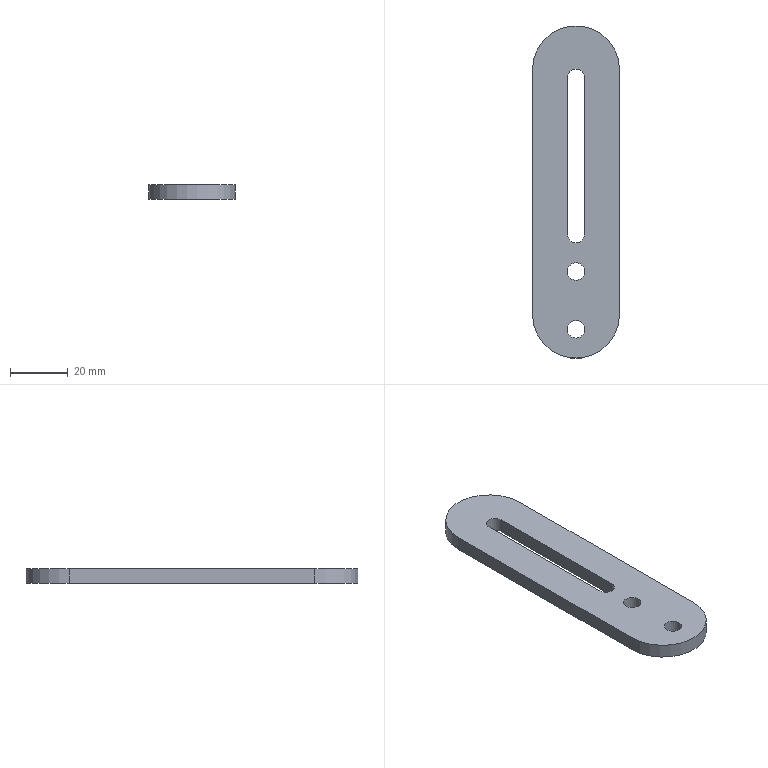Component | NX | BALL_HEAD_WAIST_PLATE | 1 solid | 12 faces | box 30 x 115 x 5 mm | volume 14240 mm3 | plane 6 | cylinder 6 | commonest cylinder face diameters 6 x4 30 x2
STEP:
#1=CARTESIAN_POINT('',(0.,0.,0.));
#2=DIRECTION('',(0.,0.,1.));
#3=DIRECTION('',(1.,0.,0.));
#4=AXIS2_PLACEMENT_3D('',#1,#2,#3);
#5=CARTESIAN_POINT('',(-63.,-45.593,2.5));
#6=VERTEX_POINT('',#5);
#7=CARTESIAN_POINT('',(-63.,8.407,2.5));
#8=VERTEX_POINT('',#7);
#9=CARTESIAN_POINT('',(-63.,-48.593,2.5));
#10=DIRECTION('',(0.,1.,0.));
#11=VECTOR('',#10,1.);
#12=LINE('',#9,#11);
#13=CARTESIAN_POINT('',(-63.,-48.593,7.5));
#14=DIRECTION('',(-1.,0.,0.));
#15=DIRECTION('',(0.,0.,-1.));
#16=AXIS2_PLACEMENT_3D('',#13,#14,#15);
#17=PLANE('',#16);
#18=CARTESIAN_POINT('',(5.,0.));
#19=DIRECTION('',(0.,-1.));
#20=VECTOR('',#19,1.);
#21=LINE('',#18,#20);
#22=(GEOMETRIC_REPRESENTATION_CONTEXT(2)PARAMETRIC_REPRESENTATION_CONTEXT()REPRESENTATION_CONTEXT('',''));
#23=DEFINITIONAL_REPRESENTATION('',(#21),#22);
#24=PCURVE('',#17,#23);
#25=CARTESIAN_POINT('',(-60.,-78.593,2.5));
#26=DIRECTION('',(0.,0.,1.));
#27=DIRECTION('',(0.,-1.,0.));
#28=AXIS2_PLACEMENT_3D('',#25,#26,#27);
#29=PLANE('',#28);
#30=CARTESIAN_POINT('',(-30.,-3.));
#31=DIRECTION('',(-1.,0.));
#32=VECTOR('',#31,1.);
#33=LINE('',#30,#32);
#34=(GEOMETRIC_REPRESENTATION_CONTEXT(2)PARAMETRIC_REPRESENTATION_CONTEXT()REPRESENTATION_CONTEXT('',''));
#35=DEFINITIONAL_REPRESENTATION('',(#33),#34);
#36=PCURVE('',#29,#35);
#37=SURFACE_CURVE('',#12,(#24,#36),.PCURVE_S1.);
#38=EDGE_CURVE('',#6,#8,#37,.T.);
#39=ORIENTED_EDGE('',*,*,#38,.T.);
#40=CARTESIAN_POINT('',(-63.,8.407,7.5));
#41=VERTEX_POINT('',#40);
#42=CARTESIAN_POINT('',(-63.,8.407,7.5));
#43=DIRECTION('',(0.,0.,1.));
#44=VECTOR('',#43,1.);
#45=LINE('',#42,#44);
#46=CARTESIAN_POINT('',(0.,-57.));
#47=DIRECTION('',(-1.,0.));
#48=VECTOR('',#47,1.);
#49=LINE('',#46,#48);
#50=(GEOMETRIC_REPRESENTATION_CONTEXT(2)PARAMETRIC_REPRESENTATION_CONTEXT()REPRESENTATION_CONTEXT('',''));
#51=DEFINITIONAL_REPRESENTATION('',(#49),#50);
#52=PCURVE('',#17,#51);
#53=CARTESIAN_POINT('',(-60.,8.407,7.5));
#54=DIRECTION('',(0.,0.,1.));
#55=DIRECTION('',(0.,-1.,0.));
#56=AXIS2_PLACEMENT_3D('',#53,#54,#55);
#57=CYLINDRICAL_SURFACE('',#56,3.);
#58=CARTESIAN_POINT('',(4.712,0.));
#59=DIRECTION('',(0.,1.));
#60=VECTOR('',#59,1.);
#61=LINE('',#58,#60);
#62=(GEOMETRIC_REPRESENTATION_CONTEXT(2)PARAMETRIC_REPRESENTATION_CONTEXT()REPRESENTATION_CONTEXT('',''));
#63=DEFINITIONAL_REPRESENTATION('',(#61),#62);
#64=PCURVE('',#57,#63);
#65=SURFACE_CURVE('',#45,(#52,#64),.PCURVE_S1.);
#66=EDGE_CURVE('',#8,#41,#65,.T.);
#67=ORIENTED_EDGE('',*,*,#66,.T.);
#68=CARTESIAN_POINT('',(-63.,-45.593,7.5));
#69=VERTEX_POINT('',#68);
#70=CARTESIAN_POINT('',(-63.,-48.593,7.5));
#71=DIRECTION('',(0.,1.,0.));
#72=VECTOR('',#71,1.);
#73=LINE('',#70,#72);
#74=CARTESIAN_POINT('',(0.,0.));
#75=DIRECTION('',(0.,-1.));
#76=VECTOR('',#75,1.);
#77=LINE('',#74,#76);
#78=(GEOMETRIC_REPRESENTATION_CONTEXT(2)PARAMETRIC_REPRESENTATION_CONTEXT()REPRESENTATION_CONTEXT('',''));
#79=DEFINITIONAL_REPRESENTATION('',(#77),#78);
#80=PCURVE('',#17,#79);
#81=CARTESIAN_POINT('',(-60.,-78.593,7.5));
#82=DIRECTION('',(0.,0.,1.));
#83=DIRECTION('',(0.,-1.,0.));
#84=AXIS2_PLACEMENT_3D('',#81,#82,#83);
#85=PLANE('',#84);
#86=CARTESIAN_POINT('',(-30.,-3.));
#87=DIRECTION('',(-1.,0.));
#88=VECTOR('',#87,1.);
#89=LINE('',#86,#88);
#90=(GEOMETRIC_REPRESENTATION_CONTEXT(2)PARAMETRIC_REPRESENTATION_CONTEXT()REPRESENTATION_CONTEXT('',''));
#91=DEFINITIONAL_REPRESENTATION('',(#89),#90);
#92=PCURVE('',#85,#91);
#93=SURFACE_CURVE('',#73,(#80,#92),.PCURVE_S1.);
#94=EDGE_CURVE('',#69,#41,#93,.T.);
#95=ORIENTED_EDGE('',*,*,#94,.F.);
#96=CARTESIAN_POINT('',(-63.,-45.593,2.5));
#97=DIRECTION('',(0.,0.,-1.));
#98=VECTOR('',#97,1.);
#99=LINE('',#96,#98);
#100=CARTESIAN_POINT('',(5.,-3.));
#101=DIRECTION('',(1.,0.));
#102=VECTOR('',#101,1.);
#103=LINE('',#100,#102);
#104=(GEOMETRIC_REPRESENTATION_CONTEXT(2)PARAMETRIC_REPRESENTATION_CONTEXT()REPRESENTATION_CONTEXT('',''));
#105=DEFINITIONAL_REPRESENTATION('',(#103),#104);
#106=PCURVE('',#17,#105);
#107=CARTESIAN_POINT('',(-60.,-45.593,7.5));
#108=DIRECTION('',(0.,0.,1.));
#109=DIRECTION('',(0.,-1.,0.));
#110=AXIS2_PLACEMENT_3D('',#107,#108,#109);
#111=CYLINDRICAL_SURFACE('',#110,3.);
#112=CARTESIAN_POINT('',(4.712,-5.));
#113=DIRECTION('',(0.,-1.));
#114=VECTOR('',#113,1.);
#115=LINE('',#112,#114);
#116=(GEOMETRIC_REPRESENTATION_CONTEXT(2)PARAMETRIC_REPRESENTATION_CONTEXT()REPRESENTATION_CONTEXT('',''));
#117=DEFINITIONAL_REPRESENTATION('',(#115),#116);
#118=PCURVE('',#111,#117);
#119=SURFACE_CURVE('',#99,(#106,#118),.PCURVE_S1.);
#120=EDGE_CURVE('',#69,#6,#119,.T.);
#121=ORIENTED_EDGE('',*,*,#120,.T.);
#122=EDGE_LOOP('',(#39,#67,#95,#121));
#123=FACE_BOUND('',#122,.T.);
#124=ADVANCED_FACE('',(#123),#17,.F.);
#125=CARTESIAN_POINT('',(-45.,11.407,2.5));
#126=VERTEX_POINT('',#125);
#127=CARTESIAN_POINT('',(-45.,-73.593,2.5));
#128=VERTEX_POINT('',#127);
#129=CARTESIAN_POINT('',(-45.,26.407,2.5));
#130=DIRECTION('',(0.,-1.,0.));
#131=VECTOR('',#130,1.);
#132=LINE('',#129,#131);
#133=CARTESIAN_POINT('',(-45.,26.407,7.5));
#134=DIRECTION('',(1.,0.,0.));
#135=DIRECTION('',(0.,0.,1.));
#136=AXIS2_PLACEMENT_3D('',#133,#134,#135);
#137=PLANE('',#136);
#138=CARTESIAN_POINT('',(-5.,0.));
#139=DIRECTION('',(0.,1.));
#140=VECTOR('',#139,1.);
#141=LINE('',#138,#140);
#142=(GEOMETRIC_REPRESENTATION_CONTEXT(2)PARAMETRIC_REPRESENTATION_CONTEXT()REPRESENTATION_CONTEXT('',''));
#143=DEFINITIONAL_REPRESENTATION('',(#141),#142);
#144=PCURVE('',#137,#143);
#145=CARTESIAN_POINT('',(-105.,15.));
#146=DIRECTION('',(1.,0.));
#147=VECTOR('',#146,1.);
#148=LINE('',#145,#147);
#149=(GEOMETRIC_REPRESENTATION_CONTEXT(2)PARAMETRIC_REPRESENTATION_CONTEXT()REPRESENTATION_CONTEXT('',''));
#150=DEFINITIONAL_REPRESENTATION('',(#148),#149);
#151=PCURVE('',#29,#150);
#152=SURFACE_CURVE('',#132,(#144,#151),.PCURVE_S1.);
#153=EDGE_CURVE('',#126,#128,#152,.T.);
#154=ORIENTED_EDGE('',*,*,#153,.F.);
#155=CARTESIAN_POINT('',(-45.,11.407,7.5));
#156=VERTEX_POINT('',#155);
#157=CARTESIAN_POINT('',(-45.,11.407,7.5));
#158=DIRECTION('',(0.,0.,1.));
#159=VECTOR('',#158,1.);
#160=LINE('',#157,#159);
#161=CARTESIAN_POINT('',(0.,15.));
#162=DIRECTION('',(1.,0.));
#163=VECTOR('',#162,1.);
#164=LINE('',#161,#163);
#165=(GEOMETRIC_REPRESENTATION_CONTEXT(2)PARAMETRIC_REPRESENTATION_CONTEXT()REPRESENTATION_CONTEXT('',''));
#166=DEFINITIONAL_REPRESENTATION('',(#164),#165);
#167=PCURVE('',#137,#166);
#168=CARTESIAN_POINT('',(-60.,11.407,7.5));
#169=DIRECTION('',(0.,0.,-1.));
#170=DIRECTION('',(0.,1.,0.));
#171=AXIS2_PLACEMENT_3D('',#168,#169,#170);
#172=CYLINDRICAL_SURFACE('',#171,15.);
#173=CARTESIAN_POINT('',(7.854,0.));
#174=DIRECTION('',(0.,-1.));
#175=VECTOR('',#174,1.);
#176=LINE('',#173,#175);
#177=(GEOMETRIC_REPRESENTATION_CONTEXT(2)PARAMETRIC_REPRESENTATION_CONTEXT()REPRESENTATION_CONTEXT('',''));
#178=DEFINITIONAL_REPRESENTATION('',(#176),#177);
#179=PCURVE('',#172,#178);
#180=SURFACE_CURVE('',#160,(#167,#179),.PCURVE_S1.);
#181=EDGE_CURVE('',#126,#156,#180,.T.);
#182=ORIENTED_EDGE('',*,*,#181,.T.);
#183=CARTESIAN_POINT('',(-45.,-73.593,7.5));
#184=VERTEX_POINT('',#183);
#185=CARTESIAN_POINT('',(-45.,26.407,7.5));
#186=DIRECTION('',(0.,-1.,0.));
#187=VECTOR('',#186,1.);
#188=LINE('',#185,#187);
#189=CARTESIAN_POINT('',(0.,0.));
#190=DIRECTION('',(0.,1.));
#191=VECTOR('',#190,1.);
#192=LINE('',#189,#191);
#193=(GEOMETRIC_REPRESENTATION_CONTEXT(2)PARAMETRIC_REPRESENTATION_CONTEXT()REPRESENTATION_CONTEXT('',''));
#194=DEFINITIONAL_REPRESENTATION('',(#192),#193);
#195=PCURVE('',#137,#194);
#196=CARTESIAN_POINT('',(-105.,15.));
#197=DIRECTION('',(1.,0.));
#198=VECTOR('',#197,1.);
#199=LINE('',#196,#198);
#200=(GEOMETRIC_REPRESENTATION_CONTEXT(2)PARAMETRIC_REPRESENTATION_CONTEXT()REPRESENTATION_CONTEXT('',''));
#201=DEFINITIONAL_REPRESENTATION('',(#199),#200);
#202=PCURVE('',#85,#201);
#203=SURFACE_CURVE('',#188,(#195,#202),.PCURVE_S1.);
#204=EDGE_CURVE('',#156,#184,#203,.T.);
#205=ORIENTED_EDGE('',*,*,#204,.T.);
#206=CARTESIAN_POINT('',(-45.,-73.593,7.5));
#207=DIRECTION('',(0.,0.,-1.));
#208=VECTOR('',#207,1.);
#209=LINE('',#206,#208);
#210=CARTESIAN_POINT('',(0.,100.));
#211=DIRECTION('',(-1.,0.));
#212=VECTOR('',#211,1.);
#213=LINE('',#210,#212);
#214=(GEOMETRIC_REPRESENTATION_CONTEXT(2)PARAMETRIC_REPRESENTATION_CONTEXT()REPRESENTATION_CONTEXT('',''));
#215=DEFINITIONAL_REPRESENTATION('',(#213),#214);
#216=PCURVE('',#137,#215);
#217=CARTESIAN_POINT('',(-60.,-73.593,7.5));
#218=DIRECTION('',(0.,0.,-1.));
#219=DIRECTION('',(0.,1.,0.));
#220=AXIS2_PLACEMENT_3D('',#217,#218,#219);
#221=CYLINDRICAL_SURFACE('',#220,15.);
#222=CARTESIAN_POINT('',(1.571,0.));
#223=DIRECTION('',(0.,1.));
#224=VECTOR('',#223,1.);
#225=LINE('',#222,#224);
#226=(GEOMETRIC_REPRESENTATION_CONTEXT(2)PARAMETRIC_REPRESENTATION_CONTEXT()REPRESENTATION_CONTEXT('',''));
#227=DEFINITIONAL_REPRESENTATION('',(#225),#226);
#228=PCURVE('',#221,#227);
#229=SURFACE_CURVE('',#209,(#216,#228),.PCURVE_S1.);
#230=EDGE_CURVE('',#184,#128,#229,.T.);
#231=ORIENTED_EDGE('',*,*,#230,.T.);
#232=EDGE_LOOP('',(#154,#182,#205,#231));
#233=FACE_BOUND('',#232,.T.);
#234=ADVANCED_FACE('',(#233),#137,.T.);
#235=CARTESIAN_POINT('',(-75.,-73.593,7.5));
#236=VERTEX_POINT('',#235);
#237=CARTESIAN_POINT('',(-75.,11.407,7.5));
#238=VERTEX_POINT('',#237);
#239=CARTESIAN_POINT('',(-75.,-88.593,7.5));
#240=DIRECTION('',(-0.,1.,0.));
#241=VECTOR('',#240,1.);
#242=LINE('',#239,#241);
#243=CARTESIAN_POINT('',(-75.,-88.593,7.5));
#244=DIRECTION('',(-1.,-0.,0.));
#245=DIRECTION('',(0.,-1.,0.));
#246=AXIS2_PLACEMENT_3D('',#243,#244,#245);
#247=PLANE('',#246);
#248=CARTESIAN_POINT('',(0.,0.));
#249=DIRECTION('',(-1.,0.));
#250=VECTOR('',#249,1.);
#251=LINE('',#248,#250);
#252=(GEOMETRIC_REPRESENTATION_CONTEXT(2)PARAMETRIC_REPRESENTATION_CONTEXT()REPRESENTATION_CONTEXT('',''));
#253=DEFINITIONAL_REPRESENTATION('',(#251),#252);
#254=PCURVE('',#247,#253);
#255=CARTESIAN_POINT('',(10.,-15.));
#256=DIRECTION('',(-1.,-0.));
#257=VECTOR('',#256,1.);
#258=LINE('',#255,#257);
#259=(GEOMETRIC_REPRESENTATION_CONTEXT(2)PARAMETRIC_REPRESENTATION_CONTEXT()REPRESENTATION_CONTEXT('',''));
#260=DEFINITIONAL_REPRESENTATION('',(#258),#259);
#261=PCURVE('',#85,#260);
#262=SURFACE_CURVE('',#242,(#254,#261),.PCURVE_S1.);
#263=EDGE_CURVE('',#236,#238,#262,.T.);
#264=ORIENTED_EDGE('',*,*,#263,.T.);
#265=CARTESIAN_POINT('',(-75.,11.407,2.5));
#266=VERTEX_POINT('',#265);
#267=CARTESIAN_POINT('',(-75.,11.407,7.5));
#268=DIRECTION('',(0.,0.,-1.));
#269=VECTOR('',#268,1.);
#270=LINE('',#267,#269);
#271=CARTESIAN_POINT('',(-100.,0.));
#272=DIRECTION('',(0.,-1.));
#273=VECTOR('',#272,1.);
#274=LINE('',#271,#273);
#275=(GEOMETRIC_REPRESENTATION_CONTEXT(2)PARAMETRIC_REPRESENTATION_CONTEXT()REPRESENTATION_CONTEXT('',''));
#276=DEFINITIONAL_REPRESENTATION('',(#274),#275);
#277=PCURVE('',#247,#276);
#278=CARTESIAN_POINT('',(4.712,0.));
#279=DIRECTION('',(0.,1.));
#280=VECTOR('',#279,1.);
#281=LINE('',#278,#280);
#282=(GEOMETRIC_REPRESENTATION_CONTEXT(2)PARAMETRIC_REPRESENTATION_CONTEXT()REPRESENTATION_CONTEXT('',''));
#283=DEFINITIONAL_REPRESENTATION('',(#281),#282);
#284=PCURVE('',#172,#283);
#285=SURFACE_CURVE('',#270,(#277,#284),.PCURVE_S1.);
#286=EDGE_CURVE('',#238,#266,#285,.T.);
#287=ORIENTED_EDGE('',*,*,#286,.T.);
#288=CARTESIAN_POINT('',(-75.,-73.593,2.5));
#289=VERTEX_POINT('',#288);
#290=CARTESIAN_POINT('',(-75.,-88.593,2.5));
#291=DIRECTION('',(-0.,1.,0.));
#292=VECTOR('',#291,1.);
#293=LINE('',#290,#292);
#294=CARTESIAN_POINT('',(0.,-5.));
#295=DIRECTION('',(-1.,0.));
#296=VECTOR('',#295,1.);
#297=LINE('',#294,#296);
#298=(GEOMETRIC_REPRESENTATION_CONTEXT(2)PARAMETRIC_REPRESENTATION_CONTEXT()REPRESENTATION_CONTEXT('',''));
#299=DEFINITIONAL_REPRESENTATION('',(#297),#298);
#300=PCURVE('',#247,#299);
#301=CARTESIAN_POINT('',(10.,-15.));
#302=DIRECTION('',(-1.,-0.));
#303=VECTOR('',#302,1.);
#304=LINE('',#301,#303);
#305=(GEOMETRIC_REPRESENTATION_CONTEXT(2)PARAMETRIC_REPRESENTATION_CONTEXT()REPRESENTATION_CONTEXT('',''));
#306=DEFINITIONAL_REPRESENTATION('',(#304),#305);
#307=PCURVE('',#29,#306);
#308=SURFACE_CURVE('',#293,(#300,#307),.PCURVE_S1.);
#309=EDGE_CURVE('',#289,#266,#308,.T.);
#310=ORIENTED_EDGE('',*,*,#309,.F.);
#311=CARTESIAN_POINT('',(-75.,-73.593,7.5));
#312=DIRECTION('',(0.,0.,1.));
#313=VECTOR('',#312,1.);
#314=LINE('',#311,#313);
#315=CARTESIAN_POINT('',(-15.,0.));
#316=DIRECTION('',(0.,1.));
#317=VECTOR('',#316,1.);
#318=LINE('',#315,#317);
#319=(GEOMETRIC_REPRESENTATION_CONTEXT(2)PARAMETRIC_REPRESENTATION_CONTEXT()REPRESENTATION_CONTEXT('',''));
#320=DEFINITIONAL_REPRESENTATION('',(#318),#319);
#321=PCURVE('',#247,#320);
#322=CARTESIAN_POINT('',(4.712,0.));
#323=DIRECTION('',(0.,-1.));
#324=VECTOR('',#323,1.);
#325=LINE('',#322,#324);
#326=(GEOMETRIC_REPRESENTATION_CONTEXT(2)PARAMETRIC_REPRESENTATION_CONTEXT()REPRESENTATION_CONTEXT('',''));
#327=DEFINITIONAL_REPRESENTATION('',(#325),#326);
#328=PCURVE('',#221,#327);
#329=SURFACE_CURVE('',#314,(#321,#328),.PCURVE_S1.);
#330=EDGE_CURVE('',#289,#236,#329,.T.);
#331=ORIENTED_EDGE('',*,*,#330,.T.);
#332=EDGE_LOOP('',(#264,#287,#310,#331));
#333=FACE_BOUND('',#332,.T.);
#334=ADVANCED_FACE('',(#333),#247,.T.);
#335=CARTESIAN_POINT('',(-60.,-61.593,7.5));
#336=VERTEX_POINT('',#335);
#337=CARTESIAN_POINT('',(-60.,-58.593,7.5));
#338=DIRECTION('',(0.,0.,1.));
#339=DIRECTION('',(0.,-1.,0.));
#340=AXIS2_PLACEMENT_3D('',#337,#338,#339);
#341=CIRCLE('',#340,3.);
#342=CARTESIAN_POINT('',(-60.,-58.593,7.5));
#343=DIRECTION('',(0.,0.,-1.));
#344=DIRECTION('',(0.,1.,0.));
#345=AXIS2_PLACEMENT_3D('',#342,#343,#344);
#346=CYLINDRICAL_SURFACE('',#345,3.);
#347=CARTESIAN_POINT('',(9.425,0.));
#348=DIRECTION('',(-1.,0.));
#349=VECTOR('',#348,1.);
#350=LINE('',#347,#349);
#351=(GEOMETRIC_REPRESENTATION_CONTEXT(2)PARAMETRIC_REPRESENTATION_CONTEXT()REPRESENTATION_CONTEXT('',''));
#352=DEFINITIONAL_REPRESENTATION('',(#350),#351);
#353=PCURVE('',#346,#352);
#354=CARTESIAN_POINT('',(-20.,0.));
#355=DIRECTION('',(1.,0.));
#356=AXIS2_PLACEMENT_2D('',#354,#355);
#357=CIRCLE('',#356,3.);
#358=(GEOMETRIC_REPRESENTATION_CONTEXT(2)PARAMETRIC_REPRESENTATION_CONTEXT()REPRESENTATION_CONTEXT('',''));
#359=DEFINITIONAL_REPRESENTATION('',(#357),#358);
#360=PCURVE('',#85,#359);
#361=SURFACE_CURVE('',#341,(#353,#360),.PCURVE_S1.);
#362=EDGE_CURVE('',#336,#336,#361,.T.);
#363=ORIENTED_EDGE('',*,*,#362,.F.);
#364=CARTESIAN_POINT('',(-60.,-61.593,2.5));
#365=VERTEX_POINT('',#364);
#366=CARTESIAN_POINT('',(-60.,-61.593,7.5));
#367=CARTESIAN_POINT('',(-60.,-61.593,2.5));
#368=B_SPLINE_CURVE_WITH_KNOTS('',1,(#366,#367),.UNSPECIFIED.,.F.,.F.,(2,2),(0.,5.),.PIECEWISE_BEZIER_KNOTS.);
#369=CARTESIAN_POINT('',(9.425,0.));
#370=DIRECTION('',(0.,1.));
#371=VECTOR('',#370,1.);
#372=LINE('',#369,#371);
#373=(GEOMETRIC_REPRESENTATION_CONTEXT(2)PARAMETRIC_REPRESENTATION_CONTEXT()REPRESENTATION_CONTEXT('',''));
#374=DEFINITIONAL_REPRESENTATION('',(#372),#373);
#375=PCURVE('',#346,#374);
#376=CARTESIAN_POINT('',(3.142,0.));
#377=DIRECTION('',(0.,1.));
#378=VECTOR('',#377,1.);
#379=LINE('',#376,#378);
#380=(GEOMETRIC_REPRESENTATION_CONTEXT(2)PARAMETRIC_REPRESENTATION_CONTEXT()REPRESENTATION_CONTEXT('',''));
#381=DEFINITIONAL_REPRESENTATION('',(#379),#380);
#382=PCURVE('',#346,#381);
#383=SEAM_CURVE('',#368,(#375,#382),.PCURVE_S1.);
#384=EDGE_CURVE('',#336,#365,#383,.T.);
#385=ORIENTED_EDGE('',*,*,#384,.T.);
#386=CARTESIAN_POINT('',(-60.,-58.593,2.5));
#387=DIRECTION('',(0.,0.,1.));
#388=DIRECTION('',(0.,-1.,0.));
#389=AXIS2_PLACEMENT_3D('',#386,#387,#388);
#390=CIRCLE('',#389,3.);
#391=CARTESIAN_POINT('',(9.425,5.));
#392=DIRECTION('',(-1.,0.));
#393=VECTOR('',#392,1.);
#394=LINE('',#391,#393);
#395=(GEOMETRIC_REPRESENTATION_CONTEXT(2)PARAMETRIC_REPRESENTATION_CONTEXT()REPRESENTATION_CONTEXT('',''));
#396=DEFINITIONAL_REPRESENTATION('',(#394),#395);
#397=PCURVE('',#346,#396);
#398=CARTESIAN_POINT('',(-20.,0.));
#399=DIRECTION('',(1.,0.));
#400=AXIS2_PLACEMENT_2D('',#398,#399);
#401=CIRCLE('',#400,3.);
#402=(GEOMETRIC_REPRESENTATION_CONTEXT(2)PARAMETRIC_REPRESENTATION_CONTEXT()REPRESENTATION_CONTEXT('',''));
#403=DEFINITIONAL_REPRESENTATION('',(#401),#402);
#404=PCURVE('',#29,#403);
#405=SURFACE_CURVE('',#390,(#397,#404),.PCURVE_S1.);
#406=EDGE_CURVE('',#365,#365,#405,.T.);
#407=ORIENTED_EDGE('',*,*,#406,.T.);
#408=ORIENTED_EDGE('',*,*,#384,.F.);
#409=EDGE_LOOP('',(#363,#385,#407,#408));
#410=FACE_BOUND('',#409,.F.);
#411=ADVANCED_FACE('',(#410),#346,.F.);
#412=CARTESIAN_POINT('',(-60.,-81.593,7.5));
#413=VERTEX_POINT('',#412);
#414=CARTESIAN_POINT('',(-60.,-78.593,7.5));
#415=DIRECTION('',(0.,0.,1.));
#416=DIRECTION('',(0.,-1.,0.));
#417=AXIS2_PLACEMENT_3D('',#414,#415,#416);
#418=CIRCLE('',#417,3.);
#419=CARTESIAN_POINT('',(-60.,-78.593,7.5));
#420=DIRECTION('',(0.,0.,-1.));
#421=DIRECTION('',(0.,1.,0.));
#422=AXIS2_PLACEMENT_3D('',#419,#420,#421);
#423=CYLINDRICAL_SURFACE('',#422,3.);
#424=CARTESIAN_POINT('',(9.425,0.));
#425=DIRECTION('',(-1.,0.));
#426=VECTOR('',#425,1.);
#427=LINE('',#424,#426);
#428=(GEOMETRIC_REPRESENTATION_CONTEXT(2)PARAMETRIC_REPRESENTATION_CONTEXT()REPRESENTATION_CONTEXT('',''));
#429=DEFINITIONAL_REPRESENTATION('',(#427),#428);
#430=PCURVE('',#423,#429);
#431=CARTESIAN_POINT('',(0.,0.));
#432=DIRECTION('',(1.,0.));
#433=AXIS2_PLACEMENT_2D('',#431,#432);
#434=CIRCLE('',#433,3.);
#435=(GEOMETRIC_REPRESENTATION_CONTEXT(2)PARAMETRIC_REPRESENTATION_CONTEXT()REPRESENTATION_CONTEXT('',''));
#436=DEFINITIONAL_REPRESENTATION('',(#434),#435);
#437=PCURVE('',#85,#436);
#438=SURFACE_CURVE('',#418,(#430,#437),.PCURVE_S1.);
#439=EDGE_CURVE('',#413,#413,#438,.T.);
#440=ORIENTED_EDGE('',*,*,#439,.F.);
#441=CARTESIAN_POINT('',(-60.,-81.593,2.5));
#442=VERTEX_POINT('',#441);
#443=CARTESIAN_POINT('',(-60.,-81.593,7.5));
#444=CARTESIAN_POINT('',(-60.,-81.593,2.5));
#445=B_SPLINE_CURVE_WITH_KNOTS('',1,(#443,#444),.UNSPECIFIED.,.F.,.F.,(2,2),(0.,5.),.PIECEWISE_BEZIER_KNOTS.);
#446=CARTESIAN_POINT('',(9.425,0.));
#447=DIRECTION('',(0.,1.));
#448=VECTOR('',#447,1.);
#449=LINE('',#446,#448);
#450=(GEOMETRIC_REPRESENTATION_CONTEXT(2)PARAMETRIC_REPRESENTATION_CONTEXT()REPRESENTATION_CONTEXT('',''));
#451=DEFINITIONAL_REPRESENTATION('',(#449),#450);
#452=PCURVE('',#423,#451);
#453=CARTESIAN_POINT('',(3.142,0.));
#454=DIRECTION('',(0.,1.));
#455=VECTOR('',#454,1.);
#456=LINE('',#453,#455);
#457=(GEOMETRIC_REPRESENTATION_CONTEXT(2)PARAMETRIC_REPRESENTATION_CONTEXT()REPRESENTATION_CONTEXT('',''));
#458=DEFINITIONAL_REPRESENTATION('',(#456),#457);
#459=PCURVE('',#423,#458);
#460=SEAM_CURVE('',#445,(#452,#459),.PCURVE_S1.);
#461=EDGE_CURVE('',#413,#442,#460,.T.);
#462=ORIENTED_EDGE('',*,*,#461,.T.);
#463=CARTESIAN_POINT('',(-60.,-78.593,2.5));
#464=DIRECTION('',(0.,0.,1.));
#465=DIRECTION('',(0.,-1.,0.));
#466=AXIS2_PLACEMENT_3D('',#463,#464,#465);
#467=CIRCLE('',#466,3.);
#468=CARTESIAN_POINT('',(9.425,5.));
#469=DIRECTION('',(-1.,0.));
#470=VECTOR('',#469,1.);
#471=LINE('',#468,#470);
#472=(GEOMETRIC_REPRESENTATION_CONTEXT(2)PARAMETRIC_REPRESENTATION_CONTEXT()REPRESENTATION_CONTEXT('',''));
#473=DEFINITIONAL_REPRESENTATION('',(#471),#472);
#474=PCURVE('',#423,#473);
#475=CARTESIAN_POINT('',(0.,0.));
#476=DIRECTION('',(1.,0.));
#477=AXIS2_PLACEMENT_2D('',#475,#476);
#478=CIRCLE('',#477,3.);
#479=(GEOMETRIC_REPRESENTATION_CONTEXT(2)PARAMETRIC_REPRESENTATION_CONTEXT()REPRESENTATION_CONTEXT('',''));
#480=DEFINITIONAL_REPRESENTATION('',(#478),#479);
#481=PCURVE('',#29,#480);
#482=SURFACE_CURVE('',#467,(#474,#481),.PCURVE_S1.);
#483=EDGE_CURVE('',#442,#442,#482,.T.);
#484=ORIENTED_EDGE('',*,*,#483,.T.);
#485=ORIENTED_EDGE('',*,*,#461,.F.);
#486=EDGE_LOOP('',(#440,#462,#484,#485));
#487=FACE_BOUND('',#486,.F.);
#488=ADVANCED_FACE('',(#487),#423,.F.);
#489=CARTESIAN_POINT('',(-57.,8.407,7.5));
#490=VERTEX_POINT('',#489);
#491=CARTESIAN_POINT('',(-57.,-45.593,7.5));
#492=VERTEX_POINT('',#491);
#493=CARTESIAN_POINT('',(-57.,11.407,7.5));
#494=DIRECTION('',(0.,-1.,0.));
#495=VECTOR('',#494,1.);
#496=LINE('',#493,#495);
#497=CARTESIAN_POINT('',(-57.,11.407,7.5));
#498=DIRECTION('',(1.,0.,0.));
#499=DIRECTION('',(0.,0.,1.));
#500=AXIS2_PLACEMENT_3D('',#497,#498,#499);
#501=PLANE('',#500);
#502=CARTESIAN_POINT('',(0.,0.));
#503=DIRECTION('',(0.,1.));
#504=VECTOR('',#503,1.);
#505=LINE('',#502,#504);
#506=(GEOMETRIC_REPRESENTATION_CONTEXT(2)PARAMETRIC_REPRESENTATION_CONTEXT()REPRESENTATION_CONTEXT('',''));
#507=DEFINITIONAL_REPRESENTATION('',(#505),#506);
#508=PCURVE('',#501,#507);
#509=CARTESIAN_POINT('',(-90.,3.));
#510=DIRECTION('',(1.,0.));
#511=VECTOR('',#510,1.);
#512=LINE('',#509,#511);
#513=(GEOMETRIC_REPRESENTATION_CONTEXT(2)PARAMETRIC_REPRESENTATION_CONTEXT()REPRESENTATION_CONTEXT('',''));
#514=DEFINITIONAL_REPRESENTATION('',(#512),#513);
#515=PCURVE('',#85,#514);
#516=SURFACE_CURVE('',#496,(#508,#515),.PCURVE_S1.);
#517=EDGE_CURVE('',#490,#492,#516,.T.);
#518=ORIENTED_EDGE('',*,*,#517,.F.);
#519=CARTESIAN_POINT('',(-57.,8.407,2.5));
#520=VERTEX_POINT('',#519);
#521=CARTESIAN_POINT('',(-57.,8.407,2.5));
#522=DIRECTION('',(0.,0.,-1.));
#523=VECTOR('',#522,1.);
#524=LINE('',#521,#523);
#525=CARTESIAN_POINT('',(-5.,3.));
#526=DIRECTION('',(-1.,0.));
#527=VECTOR('',#526,1.);
#528=LINE('',#525,#527);
#529=(GEOMETRIC_REPRESENTATION_CONTEXT(2)PARAMETRIC_REPRESENTATION_CONTEXT()REPRESENTATION_CONTEXT('',''));
#530=DEFINITIONAL_REPRESENTATION('',(#528),#529);
#531=PCURVE('',#501,#530);
#532=CARTESIAN_POINT('',(1.571,-5.));
#533=DIRECTION('',(0.,-1.));
#534=VECTOR('',#533,1.);
#535=LINE('',#532,#534);
#536=(GEOMETRIC_REPRESENTATION_CONTEXT(2)PARAMETRIC_REPRESENTATION_CONTEXT()REPRESENTATION_CONTEXT('',''));
#537=DEFINITIONAL_REPRESENTATION('',(#535),#536);
#538=PCURVE('',#57,#537);
#539=SURFACE_CURVE('',#524,(#531,#538),.PCURVE_S1.);
#540=EDGE_CURVE('',#490,#520,#539,.T.);
#541=ORIENTED_EDGE('',*,*,#540,.T.);
#542=CARTESIAN_POINT('',(-57.,-45.593,2.5));
#543=VERTEX_POINT('',#542);
#544=CARTESIAN_POINT('',(-57.,11.407,2.5));
#545=DIRECTION('',(0.,-1.,0.));
#546=VECTOR('',#545,1.);
#547=LINE('',#544,#546);
#548=CARTESIAN_POINT('',(-5.,0.));
#549=DIRECTION('',(0.,1.));
#550=VECTOR('',#549,1.);
#551=LINE('',#548,#550);
#552=(GEOMETRIC_REPRESENTATION_CONTEXT(2)PARAMETRIC_REPRESENTATION_CONTEXT()REPRESENTATION_CONTEXT('',''));
#553=DEFINITIONAL_REPRESENTATION('',(#551),#552);
#554=PCURVE('',#501,#553);
#555=CARTESIAN_POINT('',(-90.,3.));
#556=DIRECTION('',(1.,0.));
#557=VECTOR('',#556,1.);
#558=LINE('',#555,#557);
#559=(GEOMETRIC_REPRESENTATION_CONTEXT(2)PARAMETRIC_REPRESENTATION_CONTEXT()REPRESENTATION_CONTEXT('',''));
#560=DEFINITIONAL_REPRESENTATION('',(#558),#559);
#561=PCURVE('',#29,#560);
#562=SURFACE_CURVE('',#547,(#554,#561),.PCURVE_S1.);
#563=EDGE_CURVE('',#520,#543,#562,.T.);
#564=ORIENTED_EDGE('',*,*,#563,.T.);
#565=CARTESIAN_POINT('',(-57.,-45.593,7.5));
#566=DIRECTION('',(0.,0.,1.));
#567=VECTOR('',#566,1.);
#568=LINE('',#565,#567);
#569=CARTESIAN_POINT('',(0.,57.));
#570=DIRECTION('',(1.,0.));
#571=VECTOR('',#570,1.);
#572=LINE('',#569,#571);
#573=(GEOMETRIC_REPRESENTATION_CONTEXT(2)PARAMETRIC_REPRESENTATION_CONTEXT()REPRESENTATION_CONTEXT('',''));
#574=DEFINITIONAL_REPRESENTATION('',(#572),#573);
#575=PCURVE('',#501,#574);
#576=CARTESIAN_POINT('',(7.854,0.));
#577=DIRECTION('',(0.,1.));
#578=VECTOR('',#577,1.);
#579=LINE('',#576,#578);
#580=(GEOMETRIC_REPRESENTATION_CONTEXT(2)PARAMETRIC_REPRESENTATION_CONTEXT()REPRESENTATION_CONTEXT('',''));
#581=DEFINITIONAL_REPRESENTATION('',(#579),#580);
#582=PCURVE('',#111,#581);
#583=SURFACE_CURVE('',#568,(#575,#582),.PCURVE_S1.);
#584=EDGE_CURVE('',#543,#492,#583,.T.);
#585=ORIENTED_EDGE('',*,*,#584,.T.);
#586=EDGE_LOOP('',(#518,#541,#564,#585));
#587=FACE_BOUND('',#586,.T.);
#588=ADVANCED_FACE('',(#587),#501,.F.);
#589=CARTESIAN_POINT('',(-60.,11.407,7.5));
#590=DIRECTION('',(0.,0.,1.));
#591=DIRECTION('',(0.,-1.,0.));
#592=AXIS2_PLACEMENT_3D('',#589,#590,#591);
#593=CIRCLE('',#592,15.);
#594=CARTESIAN_POINT('',(-90.,0.));
#595=DIRECTION('',(1.,0.));
#596=AXIS2_PLACEMENT_2D('',#594,#595);
#597=CIRCLE('',#596,15.);
#598=(GEOMETRIC_REPRESENTATION_CONTEXT(2)PARAMETRIC_REPRESENTATION_CONTEXT()REPRESENTATION_CONTEXT('',''));
#599=DEFINITIONAL_REPRESENTATION('',(#597),#598);
#600=PCURVE('',#85,#599);
#601=CARTESIAN_POINT('',(9.425,0.));
#602=DIRECTION('',(-1.,0.));
#603=VECTOR('',#602,1.);
#604=LINE('',#601,#603);
#605=(GEOMETRIC_REPRESENTATION_CONTEXT(2)PARAMETRIC_REPRESENTATION_CONTEXT()REPRESENTATION_CONTEXT('',''));
#606=DEFINITIONAL_REPRESENTATION('',(#604),#605);
#607=PCURVE('',#172,#606);
#608=SURFACE_CURVE('',#593,(#600,#607),.PCURVE_S1.);
#609=EDGE_CURVE('',#156,#238,#608,.T.);
#610=ORIENTED_EDGE('',*,*,#609,.T.);
#611=ORIENTED_EDGE('',*,*,#263,.F.);
#612=CARTESIAN_POINT('',(-60.,-73.593,7.5));
#613=DIRECTION('',(0.,0.,1.));
#614=DIRECTION('',(0.,-1.,0.));
#615=AXIS2_PLACEMENT_3D('',#612,#613,#614);
#616=CIRCLE('',#615,15.);
#617=CARTESIAN_POINT('',(-5.,0.));
#618=DIRECTION('',(1.,0.));
#619=AXIS2_PLACEMENT_2D('',#617,#618);
#620=CIRCLE('',#619,15.);
#621=(GEOMETRIC_REPRESENTATION_CONTEXT(2)PARAMETRIC_REPRESENTATION_CONTEXT()REPRESENTATION_CONTEXT('',''));
#622=DEFINITIONAL_REPRESENTATION('',(#620),#621);
#623=PCURVE('',#85,#622);
#624=CARTESIAN_POINT('',(9.425,0.));
#625=DIRECTION('',(-1.,0.));
#626=VECTOR('',#625,1.);
#627=LINE('',#624,#626);
#628=(GEOMETRIC_REPRESENTATION_CONTEXT(2)PARAMETRIC_REPRESENTATION_CONTEXT()REPRESENTATION_CONTEXT('',''));
#629=DEFINITIONAL_REPRESENTATION('',(#627),#628);
#630=PCURVE('',#221,#629);
#631=SURFACE_CURVE('',#616,(#623,#630),.PCURVE_S1.);
#632=EDGE_CURVE('',#236,#184,#631,.T.);
#633=ORIENTED_EDGE('',*,*,#632,.T.);
#634=ORIENTED_EDGE('',*,*,#204,.F.);
#635=EDGE_LOOP('',(#610,#611,#633,#634));
#636=FACE_BOUND('',#635,.T.);
#637=ORIENTED_EDGE('',*,*,#439,.F.);
#638=EDGE_LOOP('',(#637));
#639=FACE_BOUND('',#638,.T.);
#640=ORIENTED_EDGE('',*,*,#362,.F.);
#641=EDGE_LOOP('',(#640));
#642=FACE_BOUND('',#641,.T.);
#643=ORIENTED_EDGE('',*,*,#94,.T.);
#644=CARTESIAN_POINT('',(-60.,8.407,7.5));
#645=DIRECTION('',(0.,0.,-1.));
#646=DIRECTION('',(0.,-1.,0.));
#647=AXIS2_PLACEMENT_3D('',#644,#645,#646);
#648=CIRCLE('',#647,3.);
#649=CARTESIAN_POINT('',(-84.,0.));
#650=CARTESIAN_POINT('',(-84.,-5.196));
#651=CARTESIAN_POINT('',(-88.5,-2.598));
#652=CARTESIAN_POINT('',(-93.,-0.));
#653=CARTESIAN_POINT('',(-88.5,2.598));
#654=CARTESIAN_POINT('',(-84.,5.196));
#655=CARTESIAN_POINT('',(-84.,0.));
#656=(BOUNDED_CURVE()B_SPLINE_CURVE(2,(#649,#650,#651,#652,#653,#654,#655),.UNSPECIFIED.,.T.,.F.)B_SPLINE_CURVE_WITH_KNOTS((1,2,2,2,2,1),(-2.094,0.,2.094,4.189,6.283,8.378),.UNSPECIFIED.)CURVE()GEOMETRIC_REPRESENTATION_ITEM()RATIONAL_B_SPLINE_CURVE((1.,0.5,1.,0.5,1.,0.5,1.))REPRESENTATION_ITEM(''));
#657=(GEOMETRIC_REPRESENTATION_CONTEXT(2)PARAMETRIC_REPRESENTATION_CONTEXT()REPRESENTATION_CONTEXT('',''));
#658=DEFINITIONAL_REPRESENTATION('',(#656),#657);
#659=PCURVE('',#85,#658);
#660=CARTESIAN_POINT('',(6.283,0.));
#661=DIRECTION('',(-1.,0.));
#662=VECTOR('',#661,1.);
#663=LINE('',#660,#662);
#664=(GEOMETRIC_REPRESENTATION_CONTEXT(2)PARAMETRIC_REPRESENTATION_CONTEXT()REPRESENTATION_CONTEXT('',''));
#665=DEFINITIONAL_REPRESENTATION('',(#663),#664);
#666=PCURVE('',#57,#665);
#667=SURFACE_CURVE('',#648,(#659,#666),.PCURVE_S1.);
#668=EDGE_CURVE('',#41,#490,#667,.T.);
#669=ORIENTED_EDGE('',*,*,#668,.T.);
#670=ORIENTED_EDGE('',*,*,#517,.T.);
#671=CARTESIAN_POINT('',(-60.,-45.593,7.5));
#672=DIRECTION('',(0.,0.,-1.));
#673=DIRECTION('',(0.,-1.,0.));
#674=AXIS2_PLACEMENT_3D('',#671,#672,#673);
#675=CIRCLE('',#674,3.);
#676=CARTESIAN_POINT('',(-30.,0.));
#677=CARTESIAN_POINT('',(-30.,-5.196));
#678=CARTESIAN_POINT('',(-34.5,-2.598));
#679=CARTESIAN_POINT('',(-39.,-0.));
#680=CARTESIAN_POINT('',(-34.5,2.598));
#681=CARTESIAN_POINT('',(-30.,5.196));
#682=CARTESIAN_POINT('',(-30.,0.));
#683=(BOUNDED_CURVE()B_SPLINE_CURVE(2,(#676,#677,#678,#679,#680,#681,#682),.UNSPECIFIED.,.T.,.F.)B_SPLINE_CURVE_WITH_KNOTS((1,2,2,2,2,1),(-2.094,0.,2.094,4.189,6.283,8.378),.UNSPECIFIED.)CURVE()GEOMETRIC_REPRESENTATION_ITEM()RATIONAL_B_SPLINE_CURVE((1.,0.5,1.,0.5,1.,0.5,1.))REPRESENTATION_ITEM(''));
#684=(GEOMETRIC_REPRESENTATION_CONTEXT(2)PARAMETRIC_REPRESENTATION_CONTEXT()REPRESENTATION_CONTEXT('',''));
#685=DEFINITIONAL_REPRESENTATION('',(#683),#684);
#686=PCURVE('',#85,#685);
#687=CARTESIAN_POINT('',(12.566,0.));
#688=DIRECTION('',(-1.,0.));
#689=VECTOR('',#688,1.);
#690=LINE('',#687,#689);
#691=(GEOMETRIC_REPRESENTATION_CONTEXT(2)PARAMETRIC_REPRESENTATION_CONTEXT()REPRESENTATION_CONTEXT('',''));
#692=DEFINITIONAL_REPRESENTATION('',(#690),#691);
#693=PCURVE('',#111,#692);
#694=SURFACE_CURVE('',#675,(#686,#693),.PCURVE_S1.);
#695=EDGE_CURVE('',#492,#69,#694,.T.);
#696=ORIENTED_EDGE('',*,*,#695,.T.);
#697=EDGE_LOOP('',(#643,#669,#670,#696));
#698=FACE_BOUND('',#697,.T.);
#699=ADVANCED_FACE('',(#636,#639,#642,#698),#85,.T.);
#700=ORIENTED_EDGE('',*,*,#309,.T.);
#701=CARTESIAN_POINT('',(-60.,11.407,2.5));
#702=DIRECTION('',(0.,0.,-1.));
#703=DIRECTION('',(0.,-1.,0.));
#704=AXIS2_PLACEMENT_3D('',#701,#702,#703);
#705=CIRCLE('',#704,15.);
#706=CARTESIAN_POINT('',(-75.,0.));
#707=CARTESIAN_POINT('',(-75.,-25.981));
#708=CARTESIAN_POINT('',(-97.5,-12.99));
#709=CARTESIAN_POINT('',(-120.,-0.));
#710=CARTESIAN_POINT('',(-97.5,12.99));
#711=CARTESIAN_POINT('',(-75.,25.981));
#712=CARTESIAN_POINT('',(-75.,0.));
#713=(BOUNDED_CURVE()B_SPLINE_CURVE(2,(#706,#707,#708,#709,#710,#711,#712),.UNSPECIFIED.,.T.,.F.)B_SPLINE_CURVE_WITH_KNOTS((1,2,2,2,2,1),(-2.094,0.,2.094,4.189,6.283,8.378),.UNSPECIFIED.)CURVE()GEOMETRIC_REPRESENTATION_ITEM()RATIONAL_B_SPLINE_CURVE((1.,0.5,1.,0.5,1.,0.5,1.))REPRESENTATION_ITEM(''));
#714=(GEOMETRIC_REPRESENTATION_CONTEXT(2)PARAMETRIC_REPRESENTATION_CONTEXT()REPRESENTATION_CONTEXT('',''));
#715=DEFINITIONAL_REPRESENTATION('',(#713),#714);
#716=PCURVE('',#29,#715);
#717=CARTESIAN_POINT('',(3.142,5.));
#718=DIRECTION('',(1.,0.));
#719=VECTOR('',#718,1.);
#720=LINE('',#717,#719);
#721=(GEOMETRIC_REPRESENTATION_CONTEXT(2)PARAMETRIC_REPRESENTATION_CONTEXT()REPRESENTATION_CONTEXT('',''));
#722=DEFINITIONAL_REPRESENTATION('',(#720),#721);
#723=PCURVE('',#172,#722);
#724=SURFACE_CURVE('',#705,(#716,#723),.PCURVE_S1.);
#725=EDGE_CURVE('',#266,#126,#724,.T.);
#726=ORIENTED_EDGE('',*,*,#725,.T.);
#727=ORIENTED_EDGE('',*,*,#153,.T.);
#728=CARTESIAN_POINT('',(-60.,-73.593,2.5));
#729=DIRECTION('',(0.,0.,-1.));
#730=DIRECTION('',(0.,-1.,0.));
#731=AXIS2_PLACEMENT_3D('',#728,#729,#730);
#732=CIRCLE('',#731,15.);
#733=CARTESIAN_POINT('',(10.,0.));
#734=CARTESIAN_POINT('',(10.,-25.981));
#735=CARTESIAN_POINT('',(-12.5,-12.99));
#736=CARTESIAN_POINT('',(-35.,-0.));
#737=CARTESIAN_POINT('',(-12.5,12.99));
#738=CARTESIAN_POINT('',(10.,25.981));
#739=CARTESIAN_POINT('',(10.,0.));
#740=(BOUNDED_CURVE()B_SPLINE_CURVE(2,(#733,#734,#735,#736,#737,#738,#739),.UNSPECIFIED.,.T.,.F.)B_SPLINE_CURVE_WITH_KNOTS((1,2,2,2,2,1),(-2.094,0.,2.094,4.189,6.283,8.378),.UNSPECIFIED.)CURVE()GEOMETRIC_REPRESENTATION_ITEM()RATIONAL_B_SPLINE_CURVE((1.,0.5,1.,0.5,1.,0.5,1.))REPRESENTATION_ITEM(''));
#741=(GEOMETRIC_REPRESENTATION_CONTEXT(2)PARAMETRIC_REPRESENTATION_CONTEXT()REPRESENTATION_CONTEXT('',''));
#742=DEFINITIONAL_REPRESENTATION('',(#740),#741);
#743=PCURVE('',#29,#742);
#744=CARTESIAN_POINT('',(-3.142,5.));
#745=DIRECTION('',(1.,0.));
#746=VECTOR('',#745,1.);
#747=LINE('',#744,#746);
#748=(GEOMETRIC_REPRESENTATION_CONTEXT(2)PARAMETRIC_REPRESENTATION_CONTEXT()REPRESENTATION_CONTEXT('',''));
#749=DEFINITIONAL_REPRESENTATION('',(#747),#748);
#750=PCURVE('',#221,#749);
#751=SURFACE_CURVE('',#732,(#743,#750),.PCURVE_S1.);
#752=EDGE_CURVE('',#128,#289,#751,.T.);
#753=ORIENTED_EDGE('',*,*,#752,.T.);
#754=EDGE_LOOP('',(#700,#726,#727,#753));
#755=FACE_BOUND('',#754,.T.);
#756=ORIENTED_EDGE('',*,*,#483,.T.);
#757=EDGE_LOOP('',(#756));
#758=FACE_BOUND('',#757,.T.);
#759=ORIENTED_EDGE('',*,*,#406,.T.);
#760=EDGE_LOOP('',(#759));
#761=FACE_BOUND('',#760,.T.);
#762=CARTESIAN_POINT('',(-60.,8.407,2.5));
#763=DIRECTION('',(0.,0.,1.));
#764=DIRECTION('',(0.,-1.,0.));
#765=AXIS2_PLACEMENT_3D('',#762,#763,#764);
#766=CIRCLE('',#765,3.);
#767=CARTESIAN_POINT('',(-87.,0.));
#768=DIRECTION('',(1.,0.));
#769=AXIS2_PLACEMENT_2D('',#767,#768);
#770=CIRCLE('',#769,3.);
#771=(GEOMETRIC_REPRESENTATION_CONTEXT(2)PARAMETRIC_REPRESENTATION_CONTEXT()REPRESENTATION_CONTEXT('',''));
#772=DEFINITIONAL_REPRESENTATION('',(#770),#771);
#773=PCURVE('',#29,#772);
#774=CARTESIAN_POINT('',(0.,-5.));
#775=DIRECTION('',(1.,0.));
#776=VECTOR('',#775,1.);
#777=LINE('',#774,#776);
#778=(GEOMETRIC_REPRESENTATION_CONTEXT(2)PARAMETRIC_REPRESENTATION_CONTEXT()REPRESENTATION_CONTEXT('',''));
#779=DEFINITIONAL_REPRESENTATION('',(#777),#778);
#780=PCURVE('',#57,#779);
#781=SURFACE_CURVE('',#766,(#773,#780),.PCURVE_S1.);
#782=EDGE_CURVE('',#520,#8,#781,.T.);
#783=ORIENTED_EDGE('',*,*,#782,.T.);
#784=ORIENTED_EDGE('',*,*,#38,.F.);
#785=CARTESIAN_POINT('',(-60.,-45.593,2.5));
#786=DIRECTION('',(0.,0.,1.));
#787=DIRECTION('',(0.,-1.,0.));
#788=AXIS2_PLACEMENT_3D('',#785,#786,#787);
#789=CIRCLE('',#788,3.);
#790=CARTESIAN_POINT('',(-33.,0.));
#791=DIRECTION('',(1.,0.));
#792=AXIS2_PLACEMENT_2D('',#790,#791);
#793=CIRCLE('',#792,3.);
#794=(GEOMETRIC_REPRESENTATION_CONTEXT(2)PARAMETRIC_REPRESENTATION_CONTEXT()REPRESENTATION_CONTEXT('',''));
#795=DEFINITIONAL_REPRESENTATION('',(#793),#794);
#796=PCURVE('',#29,#795);
#797=CARTESIAN_POINT('',(0.,-5.));
#798=DIRECTION('',(1.,0.));
#799=VECTOR('',#798,1.);
#800=LINE('',#797,#799);
#801=(GEOMETRIC_REPRESENTATION_CONTEXT(2)PARAMETRIC_REPRESENTATION_CONTEXT()REPRESENTATION_CONTEXT('',''));
#802=DEFINITIONAL_REPRESENTATION('',(#800),#801);
#803=PCURVE('',#111,#802);
#804=SURFACE_CURVE('',#789,(#796,#803),.PCURVE_S1.);
#805=EDGE_CURVE('',#6,#543,#804,.T.);
#806=ORIENTED_EDGE('',*,*,#805,.T.);
#807=ORIENTED_EDGE('',*,*,#563,.F.);
#808=EDGE_LOOP('',(#783,#784,#806,#807));
#809=FACE_BOUND('',#808,.T.);
#810=ADVANCED_FACE('',(#755,#758,#761,#809),#29,.F.);
#811=ORIENTED_EDGE('',*,*,#725,.F.);
#812=ORIENTED_EDGE('',*,*,#286,.F.);
#813=ORIENTED_EDGE('',*,*,#609,.F.);
#814=ORIENTED_EDGE('',*,*,#181,.F.);
#815=EDGE_LOOP('',(#811,#812,#813,#814));
#816=FACE_BOUND('',#815,.T.);
#817=ADVANCED_FACE('',(#816),#172,.T.);
#818=ORIENTED_EDGE('',*,*,#752,.F.);
#819=ORIENTED_EDGE('',*,*,#230,.F.);
#820=ORIENTED_EDGE('',*,*,#632,.F.);
#821=ORIENTED_EDGE('',*,*,#330,.F.);
#822=EDGE_LOOP('',(#818,#819,#820,#821));
#823=FACE_BOUND('',#822,.T.);
#824=ADVANCED_FACE('',(#823),#221,.T.);
#825=ORIENTED_EDGE('',*,*,#668,.T.);
#826=ORIENTED_EDGE('',*,*,#540,.T.);
#827=ORIENTED_EDGE('',*,*,#782,.T.);
#828=ORIENTED_EDGE('',*,*,#66,.T.);
#829=EDGE_LOOP('',(#825,#826,#827,#828));
#830=FACE_BOUND('',#829,.F.);
#831=ADVANCED_FACE('',(#830),#57,.F.);
#832=ORIENTED_EDGE('',*,*,#805,.T.);
#833=ORIENTED_EDGE('',*,*,#584,.T.);
#834=ORIENTED_EDGE('',*,*,#695,.T.);
#835=ORIENTED_EDGE('',*,*,#120,.T.);
#836=EDGE_LOOP('',(#832,#833,#834,#835));
#837=FACE_BOUND('',#836,.F.);
#838=ADVANCED_FACE('',(#837),#111,.F.);
#839=CLOSED_SHELL('',(#124,#234,#334,#411,#488,#588,#699,#810,#817,#824,#831,#838));
#840=MANIFOLD_SOLID_BREP('',#839);
#841=(LENGTH_UNIT()NAMED_UNIT(*)SI_UNIT(.MILLI.,.METRE.));
#842=UNCERTAINTY_MEASURE_WITH_UNIT(LENGTH_MEASURE(0.000002),#841,'','');
#843=(NAMED_UNIT(*)PLANE_ANGLE_UNIT()SI_UNIT($,.RADIAN.));
#844=(NAMED_UNIT(*)SI_UNIT($,.STERADIAN.)SOLID_ANGLE_UNIT());
#845=(GEOMETRIC_REPRESENTATION_CONTEXT(3)GLOBAL_UNCERTAINTY_ASSIGNED_CONTEXT((#842))GLOBAL_UNIT_ASSIGNED_CONTEXT((#841,#843,#844))REPRESENTATION_CONTEXT('',''));
#846=ADVANCED_BREP_SHAPE_REPRESENTATION('',(#4,#840),#845);